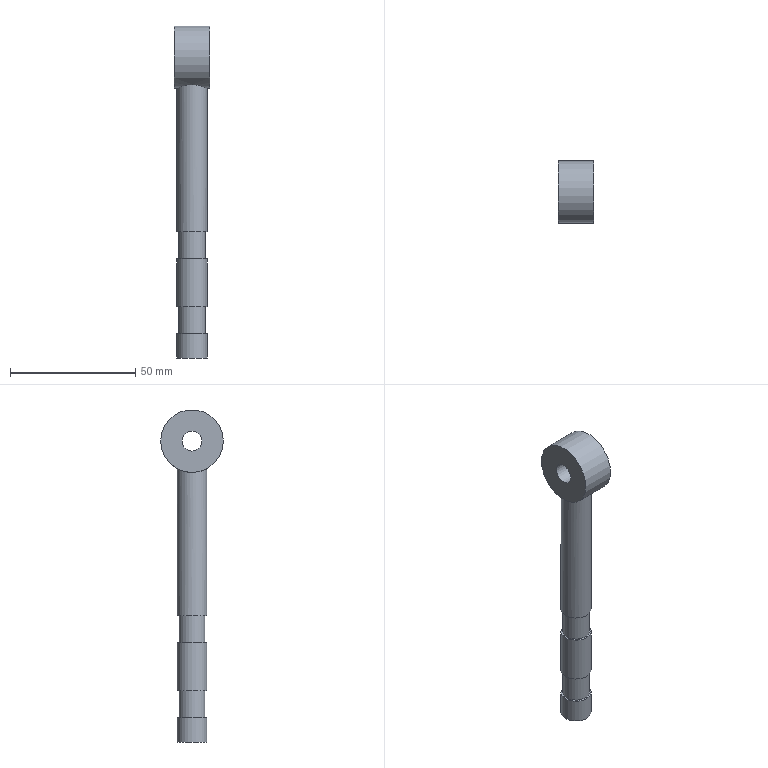Component | NX | FIXED_SCREW | 1 solid | 14 faces | box 14 x 25 x 132.5 mm | volume 17822 mm3 | cylinder 7 | plane 7 | commonest cylinder face diameters 12 x3 10.579 x2 8 x1 25 x1
STEP:
#1=CARTESIAN_POINT('',(0.,0.,0.));
#2=DIRECTION('',(0.,0.,1.));
#3=DIRECTION('',(1.,0.,0.));
#4=AXIS2_PLACEMENT_3D('',#1,#2,#3);
#5=CARTESIAN_POINT('',(566.625,96.091,-55.057));
#6=VERTEX_POINT('',#5);
#7=CARTESIAN_POINT('',(554.625,96.091,-55.057));
#8=VERTEX_POINT('',#7);
#9=CARTESIAN_POINT('',(560.625,96.091,-55.057));
#10=DIRECTION('',(0.,0.,1.));
#11=DIRECTION('',(-1.,0.,0.));
#12=AXIS2_PLACEMENT_3D('',#9,#10,#11);
#13=CIRCLE('',#12,6.);
#14=CARTESIAN_POINT('',(560.625,96.091,-94.557));
#15=DIRECTION('',(0.,0.,1.));
#16=DIRECTION('',(1.,0.,0.));
#17=AXIS2_PLACEMENT_3D('',#14,#15,#16);
#18=CYLINDRICAL_SURFACE('',#17,6.);
#19=CARTESIAN_POINT('',(-3.142,39.5));
#20=DIRECTION('',(1.,0.));
#21=VECTOR('',#20,1.);
#22=LINE('',#19,#21);
#23=(GEOMETRIC_REPRESENTATION_CONTEXT(2)PARAMETRIC_REPRESENTATION_CONTEXT()REPRESENTATION_CONTEXT('',''));
#24=DEFINITIONAL_REPRESENTATION('',(#22),#23);
#25=PCURVE('',#18,#24);
#26=CARTESIAN_POINT('',(560.625,96.091,-55.057));
#27=DIRECTION('',(0.,0.,-1.));
#28=DIRECTION('',(-1.,0.,0.));
#29=AXIS2_PLACEMENT_3D('',#26,#27,#28);
#30=PLANE('',#29);
#31=CARTESIAN_POINT('',(6.,0.));
#32=CARTESIAN_POINT('',(6.,-10.392));
#33=CARTESIAN_POINT('',(-3.,-5.196));
#34=CARTESIAN_POINT('',(-12.,-0.));
#35=CARTESIAN_POINT('',(-3.,5.196));
#36=CARTESIAN_POINT('',(6.,10.392));
#37=CARTESIAN_POINT('',(6.,0.));
#38=(BOUNDED_CURVE()B_SPLINE_CURVE(2,(#31,#32,#33,#34,#35,#36,#37),.UNSPECIFIED.,.T.,.F.)B_SPLINE_CURVE_WITH_KNOTS((1,2,2,2,2,1),(-2.094,0.,2.094,4.189,6.283,8.378),.UNSPECIFIED.)CURVE()GEOMETRIC_REPRESENTATION_ITEM()RATIONAL_B_SPLINE_CURVE((1.,0.5,1.,0.5,1.,0.5,1.))REPRESENTATION_ITEM(''));
#39=(GEOMETRIC_REPRESENTATION_CONTEXT(2)PARAMETRIC_REPRESENTATION_CONTEXT()REPRESENTATION_CONTEXT('',''));
#40=DEFINITIONAL_REPRESENTATION('',(#38),#39);
#41=PCURVE('',#30,#40);
#42=SURFACE_CURVE('',#13,(#25,#41),.PCURVE_S1.);
#43=EDGE_CURVE('',#6,#8,#42,.T.);
#44=ORIENTED_EDGE('',*,*,#43,.F.);
#45=CARTESIAN_POINT('',(566.625,96.091,-74.057));
#46=VERTEX_POINT('',#45);
#47=CARTESIAN_POINT('',(566.625,96.091,-74.057));
#48=CARTESIAN_POINT('',(566.625,96.091,-55.057));
#49=B_SPLINE_CURVE_WITH_KNOTS('',1,(#47,#48),.UNSPECIFIED.,.F.,.F.,(2,2),(20.5,39.5),.PIECEWISE_BEZIER_KNOTS.);
#50=CARTESIAN_POINT('',(0.,0.));
#51=DIRECTION('',(0.,1.));
#52=VECTOR('',#51,1.);
#53=LINE('',#50,#52);
#54=(GEOMETRIC_REPRESENTATION_CONTEXT(2)PARAMETRIC_REPRESENTATION_CONTEXT()REPRESENTATION_CONTEXT('',''));
#55=DEFINITIONAL_REPRESENTATION('',(#53),#54);
#56=PCURVE('',#18,#55);
#57=CARTESIAN_POINT('',(6.283,0.));
#58=DIRECTION('',(0.,1.));
#59=VECTOR('',#58,1.);
#60=LINE('',#57,#59);
#61=(GEOMETRIC_REPRESENTATION_CONTEXT(2)PARAMETRIC_REPRESENTATION_CONTEXT()REPRESENTATION_CONTEXT('',''));
#62=DEFINITIONAL_REPRESENTATION('',(#60),#61);
#63=PCURVE('',#18,#62);
#64=SEAM_CURVE('',#49,(#56,#63),.PCURVE_S1.);
#65=EDGE_CURVE('',#46,#6,#64,.T.);
#66=ORIENTED_EDGE('',*,*,#65,.F.);
#67=CARTESIAN_POINT('',(560.625,96.091,-74.057));
#68=DIRECTION('',(0.,0.,-1.));
#69=DIRECTION('',(1.,0.,0.));
#70=AXIS2_PLACEMENT_3D('',#67,#68,#69);
#71=CIRCLE('',#70,6.);
#72=CARTESIAN_POINT('',(6.283,20.5));
#73=DIRECTION('',(-1.,0.));
#74=VECTOR('',#73,1.);
#75=LINE('',#72,#74);
#76=(GEOMETRIC_REPRESENTATION_CONTEXT(2)PARAMETRIC_REPRESENTATION_CONTEXT()REPRESENTATION_CONTEXT('',''));
#77=DEFINITIONAL_REPRESENTATION('',(#75),#76);
#78=PCURVE('',#18,#77);
#79=CARTESIAN_POINT('',(560.625,96.091,-74.057));
#80=DIRECTION('',(0.,0.,1.));
#81=DIRECTION('',(1.,0.,0.));
#82=AXIS2_PLACEMENT_3D('',#79,#80,#81);
#83=PLANE('',#82);
#84=CARTESIAN_POINT('',(6.,0.));
#85=CARTESIAN_POINT('',(6.,-10.392));
#86=CARTESIAN_POINT('',(-3.,-5.196));
#87=CARTESIAN_POINT('',(-12.,-0.));
#88=CARTESIAN_POINT('',(-3.,5.196));
#89=CARTESIAN_POINT('',(6.,10.392));
#90=CARTESIAN_POINT('',(6.,0.));
#91=(BOUNDED_CURVE()B_SPLINE_CURVE(2,(#84,#85,#86,#87,#88,#89,#90),.UNSPECIFIED.,.T.,.F.)B_SPLINE_CURVE_WITH_KNOTS((1,2,2,2,2,1),(-2.094,0.,2.094,4.189,6.283,8.378),.UNSPECIFIED.)CURVE()GEOMETRIC_REPRESENTATION_ITEM()RATIONAL_B_SPLINE_CURVE((1.,0.5,1.,0.5,1.,0.5,1.))REPRESENTATION_ITEM(''));
#92=(GEOMETRIC_REPRESENTATION_CONTEXT(2)PARAMETRIC_REPRESENTATION_CONTEXT()REPRESENTATION_CONTEXT('',''));
#93=DEFINITIONAL_REPRESENTATION('',(#91),#92);
#94=PCURVE('',#83,#93);
#95=SURFACE_CURVE('',#71,(#78,#94),.PCURVE_S1.);
#96=EDGE_CURVE('',#46,#46,#95,.T.);
#97=ORIENTED_EDGE('',*,*,#96,.F.);
#98=ORIENTED_EDGE('',*,*,#65,.T.);
#99=CARTESIAN_POINT('',(560.625,96.091,-55.057));
#100=DIRECTION('',(0.,0.,1.));
#101=DIRECTION('',(-1.,0.,0.));
#102=AXIS2_PLACEMENT_3D('',#99,#100,#101);
#103=CIRCLE('',#102,6.);
#104=CARTESIAN_POINT('',(3.142,39.5));
#105=DIRECTION('',(1.,0.));
#106=VECTOR('',#105,1.);
#107=LINE('',#104,#106);
#108=(GEOMETRIC_REPRESENTATION_CONTEXT(2)PARAMETRIC_REPRESENTATION_CONTEXT()REPRESENTATION_CONTEXT('',''));
#109=DEFINITIONAL_REPRESENTATION('',(#107),#108);
#110=PCURVE('',#18,#109);
#111=CARTESIAN_POINT('',(6.,0.));
#112=CARTESIAN_POINT('',(6.,-10.392));
#113=CARTESIAN_POINT('',(-3.,-5.196));
#114=CARTESIAN_POINT('',(-12.,-0.));
#115=CARTESIAN_POINT('',(-3.,5.196));
#116=CARTESIAN_POINT('',(6.,10.392));
#117=CARTESIAN_POINT('',(6.,0.));
#118=(BOUNDED_CURVE()B_SPLINE_CURVE(2,(#111,#112,#113,#114,#115,#116,#117),.UNSPECIFIED.,.T.,.F.)B_SPLINE_CURVE_WITH_KNOTS((1,2,2,2,2,1),(-2.094,0.,2.094,4.189,6.283,8.378),.UNSPECIFIED.)CURVE()GEOMETRIC_REPRESENTATION_ITEM()RATIONAL_B_SPLINE_CURVE((1.,0.5,1.,0.5,1.,0.5,1.))REPRESENTATION_ITEM(''));
#119=(GEOMETRIC_REPRESENTATION_CONTEXT(2)PARAMETRIC_REPRESENTATION_CONTEXT()REPRESENTATION_CONTEXT('',''));
#120=DEFINITIONAL_REPRESENTATION('',(#118),#119);
#121=PCURVE('',#30,#120);
#122=SURFACE_CURVE('',#103,(#110,#121),.PCURVE_S1.);
#123=EDGE_CURVE('',#8,#6,#122,.T.);
#124=ORIENTED_EDGE('',*,*,#123,.F.);
#125=EDGE_LOOP('',(#44,#66,#97,#98,#124));
#126=FACE_BOUND('',#125,.T.);
#127=ADVANCED_FACE('',(#126),#18,.T.);
#128=ORIENTED_EDGE('',*,*,#96,.T.);
#129=EDGE_LOOP('',(#128));
#130=FACE_BOUND('',#129,.T.);
#131=CARTESIAN_POINT('',(565.914,96.091,-74.057));
#132=VERTEX_POINT('',#131);
#133=CARTESIAN_POINT('',(560.625,96.091,-74.057));
#134=DIRECTION('',(0.,0.,1.));
#135=DIRECTION('',(1.,0.,0.));
#136=AXIS2_PLACEMENT_3D('',#133,#134,#135);
#137=CIRCLE('',#136,5.29);
#138=CARTESIAN_POINT('',(0.,0.));
#139=DIRECTION('',(1.,0.));
#140=AXIS2_PLACEMENT_2D('',#138,#139);
#141=CIRCLE('',#140,5.29);
#142=(GEOMETRIC_REPRESENTATION_CONTEXT(2)PARAMETRIC_REPRESENTATION_CONTEXT()REPRESENTATION_CONTEXT('',''));
#143=DEFINITIONAL_REPRESENTATION('',(#141),#142);
#144=PCURVE('',#83,#143);
#145=CARTESIAN_POINT('',(560.625,96.091,-84.857));
#146=DIRECTION('',(0.,0.,1.));
#147=DIRECTION('',(1.,0.,0.));
#148=AXIS2_PLACEMENT_3D('',#145,#146,#147);
#149=CYLINDRICAL_SURFACE('',#148,5.29);
#150=CARTESIAN_POINT('',(0.,10.8));
#151=DIRECTION('',(1.,0.));
#152=VECTOR('',#151,1.);
#153=LINE('',#150,#152);
#154=(GEOMETRIC_REPRESENTATION_CONTEXT(2)PARAMETRIC_REPRESENTATION_CONTEXT()REPRESENTATION_CONTEXT('',''));
#155=DEFINITIONAL_REPRESENTATION('',(#153),#154);
#156=PCURVE('',#149,#155);
#157=SURFACE_CURVE('',#137,(#144,#156),.PCURVE_S1.);
#158=EDGE_CURVE('',#132,#132,#157,.T.);
#159=ORIENTED_EDGE('',*,*,#158,.T.);
#160=EDGE_LOOP('',(#159));
#161=FACE_BOUND('',#160,.T.);
#162=ADVANCED_FACE('',(#130,#161),#83,.F.);
#163=CARTESIAN_POINT('',(554.625,96.091,-84.857));
#164=VERTEX_POINT('',#163);
#165=CARTESIAN_POINT('',(566.625,96.091,-84.857));
#166=VERTEX_POINT('',#165);
#167=CARTESIAN_POINT('',(560.625,96.091,-84.857));
#168=DIRECTION('',(0.,0.,1.));
#169=DIRECTION('',(-1.,0.,0.));
#170=AXIS2_PLACEMENT_3D('',#167,#168,#169);
#171=CIRCLE('',#170,6.);
#172=CARTESIAN_POINT('',(560.625,96.091,-84.857));
#173=DIRECTION('',(0.,0.,-1.));
#174=DIRECTION('',(-1.,0.,0.));
#175=AXIS2_PLACEMENT_3D('',#172,#173,#174);
#176=PLANE('',#175);
#177=CARTESIAN_POINT('',(6.,0.));
#178=CARTESIAN_POINT('',(6.,-10.392));
#179=CARTESIAN_POINT('',(-3.,-5.196));
#180=CARTESIAN_POINT('',(-12.,-0.));
#181=CARTESIAN_POINT('',(-3.,5.196));
#182=CARTESIAN_POINT('',(6.,10.392));
#183=CARTESIAN_POINT('',(6.,0.));
#184=(BOUNDED_CURVE()B_SPLINE_CURVE(2,(#177,#178,#179,#180,#181,#182,#183),.UNSPECIFIED.,.T.,.F.)B_SPLINE_CURVE_WITH_KNOTS((1,2,2,2,2,1),(-2.094,0.,2.094,4.189,6.283,8.378),.UNSPECIFIED.)CURVE()GEOMETRIC_REPRESENTATION_ITEM()RATIONAL_B_SPLINE_CURVE((1.,0.5,1.,0.5,1.,0.5,1.))REPRESENTATION_ITEM(''));
#185=(GEOMETRIC_REPRESENTATION_CONTEXT(2)PARAMETRIC_REPRESENTATION_CONTEXT()REPRESENTATION_CONTEXT('',''));
#186=DEFINITIONAL_REPRESENTATION('',(#184),#185);
#187=PCURVE('',#176,#186);
#188=CARTESIAN_POINT('',(560.625,96.091,-94.557));
#189=DIRECTION('',(0.,0.,1.));
#190=DIRECTION('',(1.,0.,0.));
#191=AXIS2_PLACEMENT_3D('',#188,#189,#190);
#192=CYLINDRICAL_SURFACE('',#191,6.);
#193=CARTESIAN_POINT('',(3.142,9.7));
#194=DIRECTION('',(1.,0.));
#195=VECTOR('',#194,1.);
#196=LINE('',#193,#195);
#197=(GEOMETRIC_REPRESENTATION_CONTEXT(2)PARAMETRIC_REPRESENTATION_CONTEXT()REPRESENTATION_CONTEXT('',''));
#198=DEFINITIONAL_REPRESENTATION('',(#196),#197);
#199=PCURVE('',#192,#198);
#200=SURFACE_CURVE('',#171,(#187,#199),.PCURVE_S1.);
#201=EDGE_CURVE('',#164,#166,#200,.T.);
#202=ORIENTED_EDGE('',*,*,#201,.T.);
#203=CARTESIAN_POINT('',(560.625,96.091,-84.857));
#204=DIRECTION('',(0.,0.,1.));
#205=DIRECTION('',(-1.,0.,0.));
#206=AXIS2_PLACEMENT_3D('',#203,#204,#205);
#207=CIRCLE('',#206,6.);
#208=CARTESIAN_POINT('',(6.,0.));
#209=CARTESIAN_POINT('',(6.,-10.392));
#210=CARTESIAN_POINT('',(-3.,-5.196));
#211=CARTESIAN_POINT('',(-12.,-0.));
#212=CARTESIAN_POINT('',(-3.,5.196));
#213=CARTESIAN_POINT('',(6.,10.392));
#214=CARTESIAN_POINT('',(6.,0.));
#215=(BOUNDED_CURVE()B_SPLINE_CURVE(2,(#208,#209,#210,#211,#212,#213,#214),.UNSPECIFIED.,.T.,.F.)B_SPLINE_CURVE_WITH_KNOTS((1,2,2,2,2,1),(-2.094,0.,2.094,4.189,6.283,8.378),.UNSPECIFIED.)CURVE()GEOMETRIC_REPRESENTATION_ITEM()RATIONAL_B_SPLINE_CURVE((1.,0.5,1.,0.5,1.,0.5,1.))REPRESENTATION_ITEM(''));
#216=(GEOMETRIC_REPRESENTATION_CONTEXT(2)PARAMETRIC_REPRESENTATION_CONTEXT()REPRESENTATION_CONTEXT('',''));
#217=DEFINITIONAL_REPRESENTATION('',(#215),#216);
#218=PCURVE('',#176,#217);
#219=CARTESIAN_POINT('',(-3.142,9.7));
#220=DIRECTION('',(1.,0.));
#221=VECTOR('',#220,1.);
#222=LINE('',#219,#221);
#223=(GEOMETRIC_REPRESENTATION_CONTEXT(2)PARAMETRIC_REPRESENTATION_CONTEXT()REPRESENTATION_CONTEXT('',''));
#224=DEFINITIONAL_REPRESENTATION('',(#222),#223);
#225=PCURVE('',#192,#224);
#226=SURFACE_CURVE('',#207,(#218,#225),.PCURVE_S1.);
#227=EDGE_CURVE('',#166,#164,#226,.T.);
#228=ORIENTED_EDGE('',*,*,#227,.T.);
#229=EDGE_LOOP('',(#202,#228));
#230=FACE_BOUND('',#229,.T.);
#231=CARTESIAN_POINT('',(565.914,96.091,-84.857));
#232=VERTEX_POINT('',#231);
#233=CARTESIAN_POINT('',(560.625,96.091,-84.857));
#234=DIRECTION('',(0.,0.,-1.));
#235=DIRECTION('',(1.,0.,0.));
#236=AXIS2_PLACEMENT_3D('',#233,#234,#235);
#237=CIRCLE('',#236,5.29);
#238=CARTESIAN_POINT('',(0.,0.));
#239=DIRECTION('',(-1.,0.));
#240=AXIS2_PLACEMENT_2D('',#238,#239);
#241=CIRCLE('',#240,5.29);
#242=(GEOMETRIC_REPRESENTATION_CONTEXT(2)PARAMETRIC_REPRESENTATION_CONTEXT()REPRESENTATION_CONTEXT('',''));
#243=DEFINITIONAL_REPRESENTATION('',(#241),#242);
#244=PCURVE('',#176,#243);
#245=CARTESIAN_POINT('',(6.283,0.));
#246=DIRECTION('',(-1.,0.));
#247=VECTOR('',#246,1.);
#248=LINE('',#245,#247);
#249=(GEOMETRIC_REPRESENTATION_CONTEXT(2)PARAMETRIC_REPRESENTATION_CONTEXT()REPRESENTATION_CONTEXT('',''));
#250=DEFINITIONAL_REPRESENTATION('',(#248),#249);
#251=PCURVE('',#149,#250);
#252=SURFACE_CURVE('',#237,(#244,#251),.PCURVE_S1.);
#253=EDGE_CURVE('',#232,#232,#252,.T.);
#254=ORIENTED_EDGE('',*,*,#253,.T.);
#255=EDGE_LOOP('',(#254));
#256=FACE_BOUND('',#255,.T.);
#257=ADVANCED_FACE('',(#230,#256),#176,.F.);
#258=ORIENTED_EDGE('',*,*,#158,.F.);
#259=CARTESIAN_POINT('',(565.914,96.091,-84.857));
#260=CARTESIAN_POINT('',(565.914,96.091,-74.057));
#261=B_SPLINE_CURVE_WITH_KNOTS('',1,(#259,#260),.UNSPECIFIED.,.F.,.F.,(2,2),(0.,10.8),.PIECEWISE_BEZIER_KNOTS.);
#262=CARTESIAN_POINT('',(0.,0.));
#263=DIRECTION('',(0.,1.));
#264=VECTOR('',#263,1.);
#265=LINE('',#262,#264);
#266=(GEOMETRIC_REPRESENTATION_CONTEXT(2)PARAMETRIC_REPRESENTATION_CONTEXT()REPRESENTATION_CONTEXT('',''));
#267=DEFINITIONAL_REPRESENTATION('',(#265),#266);
#268=PCURVE('',#149,#267);
#269=CARTESIAN_POINT('',(6.283,0.));
#270=DIRECTION('',(0.,1.));
#271=VECTOR('',#270,1.);
#272=LINE('',#269,#271);
#273=(GEOMETRIC_REPRESENTATION_CONTEXT(2)PARAMETRIC_REPRESENTATION_CONTEXT()REPRESENTATION_CONTEXT('',''));
#274=DEFINITIONAL_REPRESENTATION('',(#272),#273);
#275=PCURVE('',#149,#274);
#276=SEAM_CURVE('',#261,(#268,#275),.PCURVE_S1.);
#277=EDGE_CURVE('',#232,#132,#276,.T.);
#278=ORIENTED_EDGE('',*,*,#277,.F.);
#279=ORIENTED_EDGE('',*,*,#253,.F.);
#280=ORIENTED_EDGE('',*,*,#277,.T.);
#281=EDGE_LOOP('',(#258,#278,#279,#280));
#282=FACE_BOUND('',#281,.T.);
#283=ADVANCED_FACE('',(#282),#149,.T.);
#284=CARTESIAN_POINT('',(566.625,96.091,-94.557));
#285=VERTEX_POINT('',#284);
#286=CARTESIAN_POINT('',(560.625,96.091,-94.557));
#287=DIRECTION('',(0.,0.,1.));
#288=DIRECTION('',(1.,0.,0.));
#289=AXIS2_PLACEMENT_3D('',#286,#287,#288);
#290=CIRCLE('',#289,6.);
#291=CARTESIAN_POINT('',(560.625,96.091,-94.557));
#292=DIRECTION('',(0.,0.,-1.));
#293=DIRECTION('',(-1.,0.,0.));
#294=AXIS2_PLACEMENT_3D('',#291,#292,#293);
#295=PLANE('',#294);
#296=CARTESIAN_POINT('',(-6.,0.));
#297=CARTESIAN_POINT('',(-6.,10.392));
#298=CARTESIAN_POINT('',(3.,5.196));
#299=CARTESIAN_POINT('',(12.,0.));
#300=CARTESIAN_POINT('',(3.,-5.196));
#301=CARTESIAN_POINT('',(-6.,-10.392));
#302=CARTESIAN_POINT('',(-6.,0.));
#303=(BOUNDED_CURVE()B_SPLINE_CURVE(2,(#296,#297,#298,#299,#300,#301,#302),.UNSPECIFIED.,.T.,.F.)B_SPLINE_CURVE_WITH_KNOTS((1,2,2,2,2,1),(-2.094,0.,2.094,4.189,6.283,8.378),.UNSPECIFIED.)CURVE()GEOMETRIC_REPRESENTATION_ITEM()RATIONAL_B_SPLINE_CURVE((1.,0.5,1.,0.5,1.,0.5,1.))REPRESENTATION_ITEM(''));
#304=(GEOMETRIC_REPRESENTATION_CONTEXT(2)PARAMETRIC_REPRESENTATION_CONTEXT()REPRESENTATION_CONTEXT('',''));
#305=DEFINITIONAL_REPRESENTATION('',(#303),#304);
#306=PCURVE('',#295,#305);
#307=CARTESIAN_POINT('',(0.,0.));
#308=DIRECTION('',(1.,0.));
#309=VECTOR('',#308,1.);
#310=LINE('',#307,#309);
#311=(GEOMETRIC_REPRESENTATION_CONTEXT(2)PARAMETRIC_REPRESENTATION_CONTEXT()REPRESENTATION_CONTEXT('',''));
#312=DEFINITIONAL_REPRESENTATION('',(#310),#311);
#313=PCURVE('',#192,#312);
#314=SURFACE_CURVE('',#290,(#306,#313),.PCURVE_S1.);
#315=EDGE_CURVE('',#285,#285,#314,.T.);
#316=ORIENTED_EDGE('',*,*,#315,.F.);
#317=EDGE_LOOP('',(#316));
#318=FACE_BOUND('',#317,.T.);
#319=ADVANCED_FACE('',(#318),#295,.T.);
#320=ORIENTED_EDGE('',*,*,#227,.F.);
#321=CARTESIAN_POINT('',(566.625,96.091,-94.557));
#322=CARTESIAN_POINT('',(566.625,96.091,-84.857));
#323=B_SPLINE_CURVE_WITH_KNOTS('',1,(#321,#322),.UNSPECIFIED.,.F.,.F.,(2,2),(0.,9.7),.PIECEWISE_BEZIER_KNOTS.);
#324=CARTESIAN_POINT('',(0.,0.));
#325=DIRECTION('',(0.,1.));
#326=VECTOR('',#325,1.);
#327=LINE('',#324,#326);
#328=(GEOMETRIC_REPRESENTATION_CONTEXT(2)PARAMETRIC_REPRESENTATION_CONTEXT()REPRESENTATION_CONTEXT('',''));
#329=DEFINITIONAL_REPRESENTATION('',(#327),#328);
#330=PCURVE('',#192,#329);
#331=CARTESIAN_POINT('',(6.283,0.));
#332=DIRECTION('',(0.,1.));
#333=VECTOR('',#332,1.);
#334=LINE('',#331,#333);
#335=(GEOMETRIC_REPRESENTATION_CONTEXT(2)PARAMETRIC_REPRESENTATION_CONTEXT()REPRESENTATION_CONTEXT('',''));
#336=DEFINITIONAL_REPRESENTATION('',(#334),#335);
#337=PCURVE('',#192,#336);
#338=SEAM_CURVE('',#323,(#330,#337),.PCURVE_S1.);
#339=EDGE_CURVE('',#285,#166,#338,.T.);
#340=ORIENTED_EDGE('',*,*,#339,.F.);
#341=ORIENTED_EDGE('',*,*,#315,.T.);
#342=ORIENTED_EDGE('',*,*,#339,.T.);
#343=ORIENTED_EDGE('',*,*,#201,.F.);
#344=EDGE_LOOP('',(#320,#340,#341,#342,#343));
#345=FACE_BOUND('',#344,.T.);
#346=ADVANCED_FACE('',(#345),#192,.T.);
#347=CARTESIAN_POINT('',(566.625,96.091,-44.257));
#348=VERTEX_POINT('',#347);
#349=CARTESIAN_POINT('',(560.625,96.091,-44.257));
#350=DIRECTION('',(0.,0.,-1.));
#351=DIRECTION('',(1.,0.,0.));
#352=AXIS2_PLACEMENT_3D('',#349,#350,#351);
#353=CIRCLE('',#352,6.);
#354=CARTESIAN_POINT('',(560.625,96.091,-44.257));
#355=DIRECTION('',(0.,0.,1.));
#356=DIRECTION('',(1.,0.,0.));
#357=AXIS2_PLACEMENT_3D('',#354,#355,#356);
#358=PLANE('',#357);
#359=CARTESIAN_POINT('',(6.,0.));
#360=CARTESIAN_POINT('',(6.,-10.392));
#361=CARTESIAN_POINT('',(-3.,-5.196));
#362=CARTESIAN_POINT('',(-12.,-0.));
#363=CARTESIAN_POINT('',(-3.,5.196));
#364=CARTESIAN_POINT('',(6.,10.392));
#365=CARTESIAN_POINT('',(6.,0.));
#366=(BOUNDED_CURVE()B_SPLINE_CURVE(2,(#359,#360,#361,#362,#363,#364,#365),.UNSPECIFIED.,.T.,.F.)B_SPLINE_CURVE_WITH_KNOTS((1,2,2,2,2,1),(-2.094,0.,2.094,4.189,6.283,8.378),.UNSPECIFIED.)CURVE()GEOMETRIC_REPRESENTATION_ITEM()RATIONAL_B_SPLINE_CURVE((1.,0.5,1.,0.5,1.,0.5,1.))REPRESENTATION_ITEM(''));
#367=(GEOMETRIC_REPRESENTATION_CONTEXT(2)PARAMETRIC_REPRESENTATION_CONTEXT()REPRESENTATION_CONTEXT('',''));
#368=DEFINITIONAL_REPRESENTATION('',(#366),#367);
#369=PCURVE('',#358,#368);
#370=CARTESIAN_POINT('',(560.625,96.091,-94.557));
#371=DIRECTION('',(0.,0.,1.));
#372=DIRECTION('',(1.,0.,0.));
#373=AXIS2_PLACEMENT_3D('',#370,#371,#372);
#374=CYLINDRICAL_SURFACE('',#373,6.);
#375=CARTESIAN_POINT('',(6.283,50.3));
#376=DIRECTION('',(-1.,0.));
#377=VECTOR('',#376,1.);
#378=LINE('',#375,#377);
#379=(GEOMETRIC_REPRESENTATION_CONTEXT(2)PARAMETRIC_REPRESENTATION_CONTEXT()REPRESENTATION_CONTEXT('',''));
#380=DEFINITIONAL_REPRESENTATION('',(#378),#379);
#381=PCURVE('',#374,#380);
#382=SURFACE_CURVE('',#353,(#369,#381),.PCURVE_S1.);
#383=EDGE_CURVE('',#348,#348,#382,.T.);
#384=ORIENTED_EDGE('',*,*,#383,.T.);
#385=EDGE_LOOP('',(#384));
#386=FACE_BOUND('',#385,.T.);
#387=CARTESIAN_POINT('',(565.914,96.091,-44.257));
#388=VERTEX_POINT('',#387);
#389=CARTESIAN_POINT('',(560.625,96.091,-44.257));
#390=DIRECTION('',(0.,0.,1.));
#391=DIRECTION('',(1.,0.,0.));
#392=AXIS2_PLACEMENT_3D('',#389,#390,#391);
#393=CIRCLE('',#392,5.29);
#394=CARTESIAN_POINT('',(0.,0.));
#395=DIRECTION('',(1.,0.));
#396=AXIS2_PLACEMENT_2D('',#394,#395);
#397=CIRCLE('',#396,5.29);
#398=(GEOMETRIC_REPRESENTATION_CONTEXT(2)PARAMETRIC_REPRESENTATION_CONTEXT()REPRESENTATION_CONTEXT('',''));
#399=DEFINITIONAL_REPRESENTATION('',(#397),#398);
#400=PCURVE('',#358,#399);
#401=CARTESIAN_POINT('',(560.625,96.091,-55.057));
#402=DIRECTION('',(0.,0.,1.));
#403=DIRECTION('',(1.,0.,0.));
#404=AXIS2_PLACEMENT_3D('',#401,#402,#403);
#405=CYLINDRICAL_SURFACE('',#404,5.29);
#406=CARTESIAN_POINT('',(0.,10.8));
#407=DIRECTION('',(1.,0.));
#408=VECTOR('',#407,1.);
#409=LINE('',#406,#408);
#410=(GEOMETRIC_REPRESENTATION_CONTEXT(2)PARAMETRIC_REPRESENTATION_CONTEXT()REPRESENTATION_CONTEXT('',''));
#411=DEFINITIONAL_REPRESENTATION('',(#409),#410);
#412=PCURVE('',#405,#411);
#413=SURFACE_CURVE('',#393,(#400,#412),.PCURVE_S1.);
#414=EDGE_CURVE('',#388,#388,#413,.T.);
#415=ORIENTED_EDGE('',*,*,#414,.T.);
#416=EDGE_LOOP('',(#415));
#417=FACE_BOUND('',#416,.T.);
#418=ADVANCED_FACE('',(#386,#417),#358,.F.);
#419=ORIENTED_EDGE('',*,*,#123,.T.);
#420=ORIENTED_EDGE('',*,*,#43,.T.);
#421=EDGE_LOOP('',(#419,#420));
#422=FACE_BOUND('',#421,.T.);
#423=CARTESIAN_POINT('',(565.914,96.091,-55.057));
#424=VERTEX_POINT('',#423);
#425=CARTESIAN_POINT('',(560.625,96.091,-55.057));
#426=DIRECTION('',(0.,0.,-1.));
#427=DIRECTION('',(1.,0.,0.));
#428=AXIS2_PLACEMENT_3D('',#425,#426,#427);
#429=CIRCLE('',#428,5.29);
#430=CARTESIAN_POINT('',(0.,0.));
#431=DIRECTION('',(-1.,0.));
#432=AXIS2_PLACEMENT_2D('',#430,#431);
#433=CIRCLE('',#432,5.29);
#434=(GEOMETRIC_REPRESENTATION_CONTEXT(2)PARAMETRIC_REPRESENTATION_CONTEXT()REPRESENTATION_CONTEXT('',''));
#435=DEFINITIONAL_REPRESENTATION('',(#433),#434);
#436=PCURVE('',#30,#435);
#437=CARTESIAN_POINT('',(6.283,0.));
#438=DIRECTION('',(-1.,0.));
#439=VECTOR('',#438,1.);
#440=LINE('',#437,#439);
#441=(GEOMETRIC_REPRESENTATION_CONTEXT(2)PARAMETRIC_REPRESENTATION_CONTEXT()REPRESENTATION_CONTEXT('',''));
#442=DEFINITIONAL_REPRESENTATION('',(#440),#441);
#443=PCURVE('',#405,#442);
#444=SURFACE_CURVE('',#429,(#436,#443),.PCURVE_S1.);
#445=EDGE_CURVE('',#424,#424,#444,.T.);
#446=ORIENTED_EDGE('',*,*,#445,.T.);
#447=EDGE_LOOP('',(#446));
#448=FACE_BOUND('',#447,.T.);
#449=ADVANCED_FACE('',(#422,#448),#30,.F.);
#450=ORIENTED_EDGE('',*,*,#414,.F.);
#451=CARTESIAN_POINT('',(565.914,96.091,-55.057));
#452=CARTESIAN_POINT('',(565.914,96.091,-44.257));
#453=B_SPLINE_CURVE_WITH_KNOTS('',1,(#451,#452),.UNSPECIFIED.,.F.,.F.,(2,2),(0.,10.8),.PIECEWISE_BEZIER_KNOTS.);
#454=CARTESIAN_POINT('',(0.,0.));
#455=DIRECTION('',(0.,1.));
#456=VECTOR('',#455,1.);
#457=LINE('',#454,#456);
#458=(GEOMETRIC_REPRESENTATION_CONTEXT(2)PARAMETRIC_REPRESENTATION_CONTEXT()REPRESENTATION_CONTEXT('',''));
#459=DEFINITIONAL_REPRESENTATION('',(#457),#458);
#460=PCURVE('',#405,#459);
#461=CARTESIAN_POINT('',(6.283,0.));
#462=DIRECTION('',(0.,1.));
#463=VECTOR('',#462,1.);
#464=LINE('',#461,#463);
#465=(GEOMETRIC_REPRESENTATION_CONTEXT(2)PARAMETRIC_REPRESENTATION_CONTEXT()REPRESENTATION_CONTEXT('',''));
#466=DEFINITIONAL_REPRESENTATION('',(#464),#465);
#467=PCURVE('',#405,#466);
#468=SEAM_CURVE('',#453,(#460,#467),.PCURVE_S1.);
#469=EDGE_CURVE('',#424,#388,#468,.T.);
#470=ORIENTED_EDGE('',*,*,#469,.F.);
#471=ORIENTED_EDGE('',*,*,#445,.F.);
#472=ORIENTED_EDGE('',*,*,#469,.T.);
#473=EDGE_LOOP('',(#450,#470,#471,#472));
#474=FACE_BOUND('',#473,.T.);
#475=ADVANCED_FACE('',(#474),#405,.T.);
#476=CARTESIAN_POINT('',(567.625,96.091,21.443));
#477=VERTEX_POINT('',#476);
#478=CARTESIAN_POINT('',(567.625,96.091,25.443));
#479=DIRECTION('',(1.,0.,0.));
#480=DIRECTION('',(0.,0.,-1.));
#481=AXIS2_PLACEMENT_3D('',#478,#479,#480);
#482=CIRCLE('',#481,4.);
#483=CARTESIAN_POINT('',(567.625,96.091,25.443));
#484=DIRECTION('',(-1.,0.,0.));
#485=DIRECTION('',(0.,0.,1.));
#486=AXIS2_PLACEMENT_3D('',#483,#484,#485);
#487=CYLINDRICAL_SURFACE('',#486,4.);
#488=CARTESIAN_POINT('',(9.425,0.));
#489=DIRECTION('',(-1.,0.));
#490=VECTOR('',#489,1.);
#491=LINE('',#488,#490);
#492=(GEOMETRIC_REPRESENTATION_CONTEXT(2)PARAMETRIC_REPRESENTATION_CONTEXT()REPRESENTATION_CONTEXT('',''));
#493=DEFINITIONAL_REPRESENTATION('',(#491),#492);
#494=PCURVE('',#487,#493);
#495=CARTESIAN_POINT('',(567.625,96.091,25.443));
#496=DIRECTION('',(1.,0.,0.));
#497=DIRECTION('',(0.,0.,-1.));
#498=AXIS2_PLACEMENT_3D('',#495,#496,#497);
#499=PLANE('',#498);
#500=CARTESIAN_POINT('',(0.,0.));
#501=DIRECTION('',(1.,0.));
#502=AXIS2_PLACEMENT_2D('',#500,#501);
#503=CIRCLE('',#502,4.);
#504=(GEOMETRIC_REPRESENTATION_CONTEXT(2)PARAMETRIC_REPRESENTATION_CONTEXT()REPRESENTATION_CONTEXT('',''));
#505=DEFINITIONAL_REPRESENTATION('',(#503),#504);
#506=PCURVE('',#499,#505);
#507=SURFACE_CURVE('',#482,(#494,#506),.PCURVE_S1.);
#508=EDGE_CURVE('',#477,#477,#507,.T.);
#509=ORIENTED_EDGE('',*,*,#508,.F.);
#510=CARTESIAN_POINT('',(553.625,96.091,21.443));
#511=VERTEX_POINT('',#510);
#512=CARTESIAN_POINT('',(567.625,96.091,21.443));
#513=CARTESIAN_POINT('',(553.625,96.091,21.443));
#514=B_SPLINE_CURVE_WITH_KNOTS('',1,(#512,#513),.UNSPECIFIED.,.F.,.F.,(2,2),(0.,14.),.PIECEWISE_BEZIER_KNOTS.);
#515=CARTESIAN_POINT('',(9.425,0.));
#516=DIRECTION('',(0.,1.));
#517=VECTOR('',#516,1.);
#518=LINE('',#515,#517);
#519=(GEOMETRIC_REPRESENTATION_CONTEXT(2)PARAMETRIC_REPRESENTATION_CONTEXT()REPRESENTATION_CONTEXT('',''));
#520=DEFINITIONAL_REPRESENTATION('',(#518),#519);
#521=PCURVE('',#487,#520);
#522=CARTESIAN_POINT('',(3.142,0.));
#523=DIRECTION('',(0.,1.));
#524=VECTOR('',#523,1.);
#525=LINE('',#522,#524);
#526=(GEOMETRIC_REPRESENTATION_CONTEXT(2)PARAMETRIC_REPRESENTATION_CONTEXT()REPRESENTATION_CONTEXT('',''));
#527=DEFINITIONAL_REPRESENTATION('',(#525),#526);
#528=PCURVE('',#487,#527);
#529=SEAM_CURVE('',#514,(#521,#528),.PCURVE_S1.);
#530=EDGE_CURVE('',#477,#511,#529,.T.);
#531=ORIENTED_EDGE('',*,*,#530,.T.);
#532=CARTESIAN_POINT('',(553.625,96.091,25.443));
#533=DIRECTION('',(1.,0.,0.));
#534=DIRECTION('',(0.,0.,-1.));
#535=AXIS2_PLACEMENT_3D('',#532,#533,#534);
#536=CIRCLE('',#535,4.);
#537=CARTESIAN_POINT('',(9.425,14.));
#538=DIRECTION('',(-1.,0.));
#539=VECTOR('',#538,1.);
#540=LINE('',#537,#539);
#541=(GEOMETRIC_REPRESENTATION_CONTEXT(2)PARAMETRIC_REPRESENTATION_CONTEXT()REPRESENTATION_CONTEXT('',''));
#542=DEFINITIONAL_REPRESENTATION('',(#540),#541);
#543=PCURVE('',#487,#542);
#544=CARTESIAN_POINT('',(553.625,96.091,25.443));
#545=DIRECTION('',(1.,0.,0.));
#546=DIRECTION('',(0.,0.,-1.));
#547=AXIS2_PLACEMENT_3D('',#544,#545,#546);
#548=PLANE('',#547);
#549=CARTESIAN_POINT('',(0.,0.));
#550=DIRECTION('',(1.,0.));
#551=AXIS2_PLACEMENT_2D('',#549,#550);
#552=CIRCLE('',#551,4.);
#553=(GEOMETRIC_REPRESENTATION_CONTEXT(2)PARAMETRIC_REPRESENTATION_CONTEXT()REPRESENTATION_CONTEXT('',''));
#554=DEFINITIONAL_REPRESENTATION('',(#552),#553);
#555=PCURVE('',#548,#554);
#556=SURFACE_CURVE('',#536,(#543,#555),.PCURVE_S1.);
#557=EDGE_CURVE('',#511,#511,#556,.T.);
#558=ORIENTED_EDGE('',*,*,#557,.T.);
#559=ORIENTED_EDGE('',*,*,#530,.F.);
#560=EDGE_LOOP('',(#509,#531,#558,#559));
#561=FACE_BOUND('',#560,.F.);
#562=ADVANCED_FACE('',(#561),#487,.F.);
#563=CARTESIAN_POINT('',(553.625,108.591,25.443));
#564=VERTEX_POINT('',#563);
#565=CARTESIAN_POINT('',(553.625,96.091,25.443));
#566=DIRECTION('',(1.,0.,0.));
#567=DIRECTION('',(0.,1.,0.));
#568=AXIS2_PLACEMENT_3D('',#565,#566,#567);
#569=CIRCLE('',#568,12.5);
#570=CARTESIAN_POINT('',(0.,0.));
#571=DIRECTION('',(0.,1.));
#572=AXIS2_PLACEMENT_2D('',#570,#571);
#573=CIRCLE('',#572,12.5);
#574=(GEOMETRIC_REPRESENTATION_CONTEXT(2)PARAMETRIC_REPRESENTATION_CONTEXT()REPRESENTATION_CONTEXT('',''));
#575=DEFINITIONAL_REPRESENTATION('',(#573),#574);
#576=PCURVE('',#548,#575);
#577=CARTESIAN_POINT('',(567.625,96.091,25.443));
#578=DIRECTION('',(-1.,0.,0.));
#579=DIRECTION('',(0.,0.,1.));
#580=AXIS2_PLACEMENT_3D('',#577,#578,#579);
#581=CYLINDRICAL_SURFACE('',#580,12.5);
#582=CARTESIAN_POINT('',(7.854,14.));
#583=DIRECTION('',(-1.,0.));
#584=VECTOR('',#583,1.);
#585=LINE('',#582,#584);
#586=(GEOMETRIC_REPRESENTATION_CONTEXT(2)PARAMETRIC_REPRESENTATION_CONTEXT()REPRESENTATION_CONTEXT('',''));
#587=DEFINITIONAL_REPRESENTATION('',(#585),#586);
#588=PCURVE('',#581,#587);
#589=SURFACE_CURVE('',#569,(#576,#588),.PCURVE_S1.);
#590=EDGE_CURVE('',#564,#564,#589,.T.);
#591=ORIENTED_EDGE('',*,*,#590,.F.);
#592=EDGE_LOOP('',(#591));
#593=FACE_BOUND('',#592,.T.);
#594=ORIENTED_EDGE('',*,*,#557,.T.);
#595=EDGE_LOOP('',(#594));
#596=FACE_BOUND('',#595,.T.);
#597=ADVANCED_FACE('',(#593,#596),#548,.F.);
#598=CARTESIAN_POINT('',(567.625,108.591,25.443));
#599=VERTEX_POINT('',#598);
#600=CARTESIAN_POINT('',(567.625,96.091,25.443));
#601=DIRECTION('',(1.,0.,0.));
#602=DIRECTION('',(0.,1.,0.));
#603=AXIS2_PLACEMENT_3D('',#600,#601,#602);
#604=CIRCLE('',#603,12.5);
#605=CARTESIAN_POINT('',(0.,0.));
#606=DIRECTION('',(0.,1.));
#607=AXIS2_PLACEMENT_2D('',#605,#606);
#608=CIRCLE('',#607,12.5);
#609=(GEOMETRIC_REPRESENTATION_CONTEXT(2)PARAMETRIC_REPRESENTATION_CONTEXT()REPRESENTATION_CONTEXT('',''));
#610=DEFINITIONAL_REPRESENTATION('',(#608),#609);
#611=PCURVE('',#499,#610);
#612=CARTESIAN_POINT('',(7.854,0.));
#613=DIRECTION('',(-1.,0.));
#614=VECTOR('',#613,1.);
#615=LINE('',#612,#614);
#616=(GEOMETRIC_REPRESENTATION_CONTEXT(2)PARAMETRIC_REPRESENTATION_CONTEXT()REPRESENTATION_CONTEXT('',''));
#617=DEFINITIONAL_REPRESENTATION('',(#615),#616);
#618=PCURVE('',#581,#617);
#619=SURFACE_CURVE('',#604,(#611,#618),.PCURVE_S1.);
#620=EDGE_CURVE('',#599,#599,#619,.T.);
#621=ORIENTED_EDGE('',*,*,#620,.T.);
#622=EDGE_LOOP('',(#621));
#623=FACE_BOUND('',#622,.T.);
#624=ORIENTED_EDGE('',*,*,#508,.F.);
#625=EDGE_LOOP('',(#624));
#626=FACE_BOUND('',#625,.T.);
#627=ADVANCED_FACE('',(#623,#626),#499,.T.);
#628=ORIENTED_EDGE('',*,*,#620,.F.);
#629=CARTESIAN_POINT('',(567.625,108.591,25.443));
#630=CARTESIAN_POINT('',(553.625,108.591,25.443));
#631=B_SPLINE_CURVE_WITH_KNOTS('',1,(#629,#630),.UNSPECIFIED.,.F.,.F.,(2,2),(0.,14.),.PIECEWISE_BEZIER_KNOTS.);
#632=CARTESIAN_POINT('',(7.854,0.));
#633=DIRECTION('',(0.,1.));
#634=VECTOR('',#633,1.);
#635=LINE('',#632,#634);
#636=(GEOMETRIC_REPRESENTATION_CONTEXT(2)PARAMETRIC_REPRESENTATION_CONTEXT()REPRESENTATION_CONTEXT('',''));
#637=DEFINITIONAL_REPRESENTATION('',(#635),#636);
#638=PCURVE('',#581,#637);
#639=CARTESIAN_POINT('',(1.571,0.));
#640=DIRECTION('',(0.,1.));
#641=VECTOR('',#640,1.);
#642=LINE('',#639,#641);
#643=(GEOMETRIC_REPRESENTATION_CONTEXT(2)PARAMETRIC_REPRESENTATION_CONTEXT()REPRESENTATION_CONTEXT('',''));
#644=DEFINITIONAL_REPRESENTATION('',(#642),#643);
#645=PCURVE('',#581,#644);
#646=SEAM_CURVE('',#631,(#638,#645),.PCURVE_S1.);
#647=EDGE_CURVE('',#599,#564,#646,.T.);
#648=ORIENTED_EDGE('',*,*,#647,.T.);
#649=ORIENTED_EDGE('',*,*,#590,.T.);
#650=ORIENTED_EDGE('',*,*,#647,.F.);
#651=EDGE_LOOP('',(#628,#648,#649,#650));
#652=FACE_BOUND('',#651,.T.);
#653=CARTESIAN_POINT('',(566.625,96.091,12.943));
#654=VERTEX_POINT('',#653);
#655=CARTESIAN_POINT('',(566.625,97.702,12.943));
#656=CARTESIAN_POINT('',(566.625,94.479,12.943));
#657=CARTESIAN_POINT('',(565.955,92.935,13.293));
#658=CARTESIAN_POINT('',(563.776,90.758,14.079));
#659=CARTESIAN_POINT('',(562.23,90.094,14.475));
#660=CARTESIAN_POINT('',(559.044,90.087,14.479));
#661=CARTESIAN_POINT('',(557.481,90.753,14.081));
#662=CARTESIAN_POINT('',(555.297,92.929,13.294));
#663=CARTESIAN_POINT('',(554.629,94.488,12.945));
#664=CARTESIAN_POINT('',(554.621,97.665,12.941));
#665=CARTESIAN_POINT('',(555.286,99.236,13.289));
#666=CARTESIAN_POINT('',(557.474,101.426,14.079));
#667=CARTESIAN_POINT('',(559.026,102.087,14.475));
#668=CARTESIAN_POINT('',(562.199,102.094,14.479));
#669=CARTESIAN_POINT('',(563.76,101.438,14.084));
#670=CARTESIAN_POINT('',(565.964,99.24,13.29));
#671=CARTESIAN_POINT('',(566.625,97.702,12.943));
#672=CARTESIAN_POINT('',(566.625,94.479,12.943));
#673=B_SPLINE_CURVE_WITH_KNOTS('',3,(#655,#656,#657,#658,#659,#660,#661,#662,#663,#664,#665,#666,#667,#668,#669,#670,#671,#672),.UNSPECIFIED.,.T.,.F.,(2,2,2,2,2,2,2,2,2,2,2),(-0.125,0.,0.125,0.25,0.375,0.5,0.625,0.75,0.875,1.,1.125),.UNSPECIFIED.);
#674=CARTESIAN_POINT('',(3.142,1.));
#675=CARTESIAN_POINT('',(3.165,1.));
#676=CARTESIAN_POINT('',(3.212,1.044));
#677=CARTESIAN_POINT('',(3.28,1.235));
#678=CARTESIAN_POINT('',(3.345,1.54));
#679=CARTESIAN_POINT('',(3.406,1.95));
#680=CARTESIAN_POINT('',(3.463,2.458));
#681=CARTESIAN_POINT('',(3.514,3.053));
#682=CARTESIAN_POINT('',(3.557,3.733));
#683=CARTESIAN_POINT('',(3.593,4.48));
#684=CARTESIAN_POINT('',(3.621,5.282));
#685=CARTESIAN_POINT('',(3.638,6.122));
#686=CARTESIAN_POINT('',(3.644,6.987));
#687=CARTESIAN_POINT('',(3.638,7.855));
#688=CARTESIAN_POINT('',(3.621,8.699));
#689=CARTESIAN_POINT('',(3.594,9.505));
#690=CARTESIAN_POINT('',(3.558,10.258));
#691=CARTESIAN_POINT('',(3.514,10.941));
#692=CARTESIAN_POINT('',(3.463,11.537));
#693=CARTESIAN_POINT('',(3.407,12.046));
#694=CARTESIAN_POINT('',(3.345,12.457));
#695=CARTESIAN_POINT('',(3.28,12.763));
#696=CARTESIAN_POINT('',(3.212,12.954));
#697=CARTESIAN_POINT('',(3.143,13.022));
#698=CARTESIAN_POINT('',(3.073,12.958));
#699=CARTESIAN_POINT('',(3.006,12.77));
#700=CARTESIAN_POINT('',(2.94,12.466));
#701=CARTESIAN_POINT('',(2.878,12.055));
#702=CARTESIAN_POINT('',(2.821,11.547));
#703=CARTESIAN_POINT('',(2.77,10.949));
#704=CARTESIAN_POINT('',(2.726,10.267));
#705=CARTESIAN_POINT('',(2.69,9.518));
#706=CARTESIAN_POINT('',(2.662,8.715));
#707=CARTESIAN_POINT('',(2.645,7.876));
#708=CARTESIAN_POINT('',(2.639,7.012));
#709=CARTESIAN_POINT('',(2.645,6.148));
#710=CARTESIAN_POINT('',(2.662,5.307));
#711=CARTESIAN_POINT('',(2.689,4.501));
#712=CARTESIAN_POINT('',(2.725,3.747));
#713=CARTESIAN_POINT('',(2.769,3.061));
#714=CARTESIAN_POINT('',(2.82,2.458));
#715=CARTESIAN_POINT('',(2.877,1.948));
#716=CARTESIAN_POINT('',(2.939,1.536));
#717=CARTESIAN_POINT('',(3.004,1.232));
#718=CARTESIAN_POINT('',(3.072,1.044));
#719=CARTESIAN_POINT('',(3.118,1.));
#720=CARTESIAN_POINT('',(3.142,1.));
#721=B_SPLINE_CURVE_WITH_KNOTS('',3,(#674,#675,#676,#677,#678,#679,#680,#681,#682,#683,#684,#685,#686,#687,#688,#689,#690,#691,#692,#693,#694,#695,#696,#697,#698,#699,#700,#701,#702,#703,#704,#705,#706,#707,#708,#709,#710,#711,#712,#713,#714,#715,#716,#717,#718,#719,#720),.UNSPECIFIED.,.T.,.F.,(4,1,1,1,1,1,1,1,1,1,1,1,1,1,1,1,1,1,1,1,1,1,1,1,1,1,1,1,1,1,1,1,1,1,1,1,1,1,1,1,1,1,1,1,4),(0.,0.02273,0.04545,0.06818,0.09091,0.1136,0.1364,0.1591,0.1818,0.2045,0.2273,0.25,0.2727,0.2955,0.3182,0.3409,0.3636,0.3864,0.4091,0.4318,0.4545,0.4773,0.5,0.5227,0.5455,0.5682,0.5909,0.6136,0.6364,0.6591,0.6818,0.7045,0.7273,0.75,0.7727,0.7955,0.8182,0.8409,0.8636,0.8864,0.9091,0.9318,0.9545,0.9773,1.),.QUASI_UNIFORM_KNOTS.);
#722=(GEOMETRIC_REPRESENTATION_CONTEXT(2)PARAMETRIC_REPRESENTATION_CONTEXT()REPRESENTATION_CONTEXT('',''));
#723=DEFINITIONAL_REPRESENTATION('',(#721),#722);
#724=PCURVE('',#581,#723);
#725=CARTESIAN_POINT('',(6.283,107.5));
#726=CARTESIAN_POINT('',(6.234,107.5));
#727=CARTESIAN_POINT('',(6.137,107.523));
#728=CARTESIAN_POINT('',(5.993,107.616));
#729=CARTESIAN_POINT('',(5.85,107.756));
#730=CARTESIAN_POINT('',(5.708,107.933));
#731=CARTESIAN_POINT('',(5.567,108.134));
#732=CARTESIAN_POINT('',(5.427,108.351));
#733=CARTESIAN_POINT('',(5.287,108.56));
#734=CARTESIAN_POINT('',(5.145,108.749));
#735=CARTESIAN_POINT('',(5.002,108.903));
#736=CARTESIAN_POINT('',(4.859,109.007));
#737=CARTESIAN_POINT('',(4.714,109.047));
#738=CARTESIAN_POINT('',(4.57,109.009));
#739=CARTESIAN_POINT('',(4.426,108.905));
#740=CARTESIAN_POINT('',(4.283,108.752));
#741=CARTESIAN_POINT('',(4.14,108.563));
#742=CARTESIAN_POINT('',(3.999,108.353));
#743=CARTESIAN_POINT('',(3.859,108.136));
#744=CARTESIAN_POINT('',(3.717,107.935));
#745=CARTESIAN_POINT('',(3.575,107.758));
#746=CARTESIAN_POINT('',(3.432,107.617));
#747=CARTESIAN_POINT('',(3.288,107.524));
#748=CARTESIAN_POINT('',(3.144,107.488));
#749=CARTESIAN_POINT('',(3.,107.522));
#750=CARTESIAN_POINT('',(2.856,107.614));
#751=CARTESIAN_POINT('',(2.712,107.754));
#752=CARTESIAN_POINT('',(2.569,107.931));
#753=CARTESIAN_POINT('',(2.427,108.132));
#754=CARTESIAN_POINT('',(2.286,108.35));
#755=CARTESIAN_POINT('',(2.145,108.56));
#756=CARTESIAN_POINT('',(2.003,108.749));
#757=CARTESIAN_POINT('',(1.86,108.903));
#758=CARTESIAN_POINT('',(1.717,109.007));
#759=CARTESIAN_POINT('',(1.573,109.047));
#760=CARTESIAN_POINT('',(1.429,109.009));
#761=CARTESIAN_POINT('',(1.285,108.906));
#762=CARTESIAN_POINT('',(1.142,108.753));
#763=CARTESIAN_POINT('',(0.9995,108.564));
#764=CARTESIAN_POINT('',(0.8574,108.353));
#765=CARTESIAN_POINT('',(0.716,108.134));
#766=CARTESIAN_POINT('',(0.5744,107.932));
#767=CARTESIAN_POINT('',(0.4323,107.755));
#768=CARTESIAN_POINT('',(0.2895,107.615));
#769=CARTESIAN_POINT('',(0.1457,107.523));
#770=CARTESIAN_POINT('',(0.0488,107.5));
#771=CARTESIAN_POINT('',(-0.,107.5));
#772=B_SPLINE_CURVE_WITH_KNOTS('',3,(#725,#726,#727,#728,#729,#730,#731,#732,#733,#734,#735,#736,#737,#738,#739,#740,#741,#742,#743,#744,#745,#746,#747,#748,#749,#750,#751,#752,#753,#754,#755,#756,#757,#758,#759,#760,#761,#762,#763,#764,#765,#766,#767,#768,#769,#770,#771),.UNSPECIFIED.,.F.,.F.,(4,1,1,1,1,1,1,1,1,1,1,1,1,1,1,1,1,1,1,1,1,1,1,1,1,1,1,1,1,1,1,1,1,1,1,1,1,1,1,1,1,1,1,1,4),(0.,0.02273,0.04545,0.06818,0.09091,0.1136,0.1364,0.1591,0.1818,0.2045,0.2273,0.25,0.2727,0.2955,0.3182,0.3409,0.3636,0.3864,0.4091,0.4318,0.4545,0.4773,0.5,0.5227,0.5455,0.5682,0.5909,0.6136,0.6364,0.6591,0.6818,0.7045,0.7273,0.75,0.7727,0.7955,0.8182,0.8409,0.8636,0.8864,0.9091,0.9318,0.9545,0.9773,1.),.QUASI_UNIFORM_KNOTS.);
#773=(GEOMETRIC_REPRESENTATION_CONTEXT(2)PARAMETRIC_REPRESENTATION_CONTEXT()REPRESENTATION_CONTEXT('',''));
#774=DEFINITIONAL_REPRESENTATION('',(#772),#773);
#775=PCURVE('',#374,#774);
#776=SURFACE_CURVE('',#673,(#724,#775),.PCURVE_S1.);
#777=EDGE_CURVE('',#654,#654,#776,.T.);
#778=ORIENTED_EDGE('',*,*,#777,.F.);
#779=EDGE_LOOP('',(#778));
#780=FACE_BOUND('',#779,.T.);
#781=ADVANCED_FACE('',(#652,#780),#581,.T.);
#782=ORIENTED_EDGE('',*,*,#383,.F.);
#783=CARTESIAN_POINT('',(566.625,96.091,-44.257));
#784=CARTESIAN_POINT('',(566.625,96.091,12.943));
#785=B_SPLINE_CURVE_WITH_KNOTS('',1,(#783,#784),.UNSPECIFIED.,.F.,.F.,(2,2),(50.3,107.5),.PIECEWISE_BEZIER_KNOTS.);
#786=CARTESIAN_POINT('',(6.283,0.));
#787=DIRECTION('',(0.,1.));
#788=VECTOR('',#787,1.);
#789=LINE('',#786,#788);
#790=(GEOMETRIC_REPRESENTATION_CONTEXT(2)PARAMETRIC_REPRESENTATION_CONTEXT()REPRESENTATION_CONTEXT('',''));
#791=DEFINITIONAL_REPRESENTATION('',(#789),#790);
#792=PCURVE('',#374,#791);
#793=CARTESIAN_POINT('',(0.,0.));
#794=DIRECTION('',(0.,1.));
#795=VECTOR('',#794,1.);
#796=LINE('',#793,#795);
#797=(GEOMETRIC_REPRESENTATION_CONTEXT(2)PARAMETRIC_REPRESENTATION_CONTEXT()REPRESENTATION_CONTEXT('',''));
#798=DEFINITIONAL_REPRESENTATION('',(#796),#797);
#799=PCURVE('',#374,#798);
#800=SEAM_CURVE('',#785,(#792,#799),.PCURVE_S1.);
#801=EDGE_CURVE('',#348,#654,#800,.T.);
#802=ORIENTED_EDGE('',*,*,#801,.T.);
#803=ORIENTED_EDGE('',*,*,#777,.T.);
#804=ORIENTED_EDGE('',*,*,#801,.F.);
#805=EDGE_LOOP('',(#782,#802,#803,#804));
#806=FACE_BOUND('',#805,.T.);
#807=ADVANCED_FACE('',(#806),#374,.T.);
#808=CLOSED_SHELL('',(#127,#162,#257,#283,#319,#346,#418,#449,#475,#562,#597,#627,#781,#807));
#809=MANIFOLD_SOLID_BREP('',#808);
#810=(LENGTH_UNIT()NAMED_UNIT(*)SI_UNIT(.MILLI.,.METRE.));
#811=UNCERTAINTY_MEASURE_WITH_UNIT(LENGTH_MEASURE(0.0005),#810,'','');
#812=(NAMED_UNIT(*)PLANE_ANGLE_UNIT()SI_UNIT($,.RADIAN.));
#813=(NAMED_UNIT(*)SI_UNIT($,.STERADIAN.)SOLID_ANGLE_UNIT());
#814=(GEOMETRIC_REPRESENTATION_CONTEXT(3)GLOBAL_UNCERTAINTY_ASSIGNED_CONTEXT((#811))GLOBAL_UNIT_ASSIGNED_CONTEXT((#810,#812,#813))REPRESENTATION_CONTEXT('',''));
#815=ADVANCED_BREP_SHAPE_REPRESENTATION('',(#4,#809),#814);